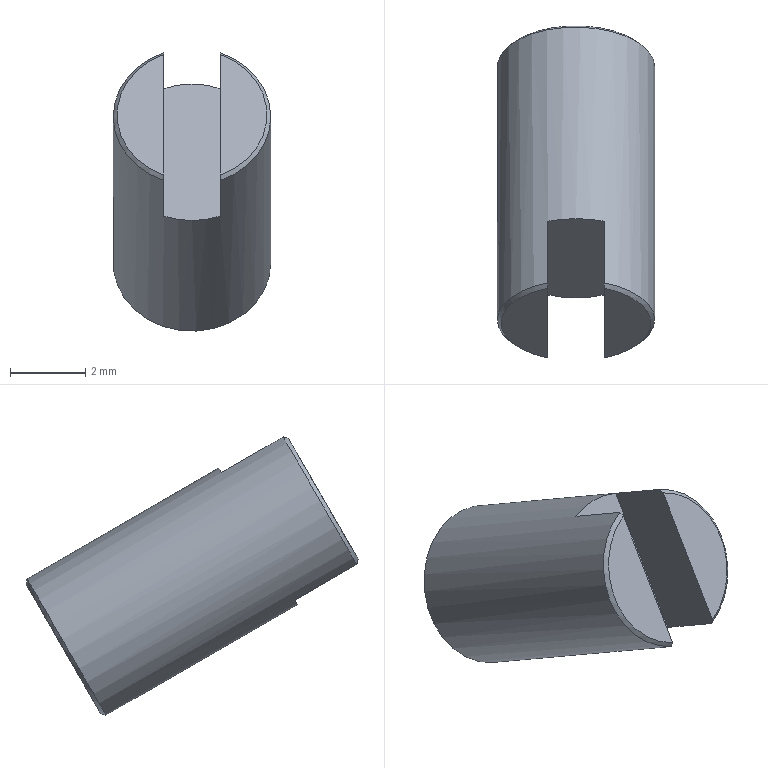Component | NX | 14_AIR_PLUG_2 | 1 solid | 10 faces | box 4.2 x 8.86 x 7.42 mm | volume 98 mm3 | plane 6 | cone 3 | cylinder 1 | commonest cylinder face diameters 4.2 x1
STEP:
#1=CARTESIAN_POINT('',(0.,0.,0.));
#2=DIRECTION('',(0.,0.,1.));
#3=DIRECTION('',(1.,0.,0.));
#4=AXIS2_PLACEMENT_3D('',#1,#2,#3);
#5=CARTESIAN_POINT('',(-58.334,-83.371,-220.899));
#6=VERTEX_POINT('',#5);
#7=CARTESIAN_POINT('',(-58.334,-85.225,-224.111));
#8=VERTEX_POINT('',#7);
#9=CARTESIAN_POINT('',(-58.334,-84.298,-222.505));
#10=DIRECTION('',(0.,-0.5,-0.866));
#11=VECTOR('',#10,1.);
#12=LINE('',#9,#11);
#13=CARTESIAN_POINT('',(-59.084,-84.298,-222.505));
#14=DIRECTION('',(0.,-0.866,0.5));
#15=DIRECTION('',(1.,0.,0.));
#16=AXIS2_PLACEMENT_3D('',#13,#14,#15);
#17=PLANE('',#16);
#18=CARTESIAN_POINT('',(0.75,0.));
#19=DIRECTION('',(0.,-1.));
#20=VECTOR('',#19,1.);
#21=LINE('',#18,#20);
#22=(GEOMETRIC_REPRESENTATION_CONTEXT(2)PARAMETRIC_REPRESENTATION_CONTEXT()REPRESENTATION_CONTEXT('',''));
#23=DEFINITIONAL_REPRESENTATION('',(#21),#22);
#24=PCURVE('',#17,#23);
#25=CARTESIAN_POINT('',(-58.334,-81.316,-221.34));
#26=DIRECTION('',(-1.,-0.,-0.));
#27=DIRECTION('',(0.,-0.5,-0.866));
#28=AXIS2_PLACEMENT_3D('',#25,#26,#27);
#29=PLANE('',#28);
#30=CARTESIAN_POINT('',(2.5,2.));
#31=DIRECTION('',(1.,0.));
#32=VECTOR('',#31,1.);
#33=LINE('',#30,#32);
#34=(GEOMETRIC_REPRESENTATION_CONTEXT(2)PARAMETRIC_REPRESENTATION_CONTEXT()REPRESENTATION_CONTEXT('',''));
#35=DEFINITIONAL_REPRESENTATION('',(#33),#34);
#36=PCURVE('',#29,#35);
#37=SURFACE_CURVE('',#12,(#24,#36),.PCURVE_S1.);
#38=EDGE_CURVE('',#6,#8,#37,.T.);
#39=ORIENTED_EDGE('',*,*,#38,.T.);
#40=CARTESIAN_POINT('',(-59.084,-84.298,-222.505));
#41=DIRECTION('',(0.,-0.866,0.5));
#42=DIRECTION('',(1.,0.,0.));
#43=AXIS2_PLACEMENT_3D('',#40,#41,#42);
#44=CIRCLE('',#43,2.);
#45=CARTESIAN_POINT('',(0.,0.));
#46=DIRECTION('',(1.,0.));
#47=AXIS2_PLACEMENT_2D('',#45,#46);
#48=CIRCLE('',#47,2.);
#49=(GEOMETRIC_REPRESENTATION_CONTEXT(2)PARAMETRIC_REPRESENTATION_CONTEXT()REPRESENTATION_CONTEXT('',''));
#50=DEFINITIONAL_REPRESENTATION('',(#48),#49);
#51=PCURVE('',#17,#50);
#52=CARTESIAN_POINT('',(-59.084,-83.865,-222.755));
#53=DIRECTION('',(0.,0.866,-0.5));
#54=DIRECTION('',(-1.,-0.,-0.));
#55=AXIS2_PLACEMENT_3D('',#52,#53,#54);
#56=CONICAL_SURFACE('',#55,2.5,0.7854);
#57=CARTESIAN_POINT('',(9.425,-0.5));
#58=DIRECTION('',(-1.,-0.));
#59=VECTOR('',#58,1.);
#60=LINE('',#57,#59);
#61=(GEOMETRIC_REPRESENTATION_CONTEXT(2)PARAMETRIC_REPRESENTATION_CONTEXT()REPRESENTATION_CONTEXT('',''));
#62=DEFINITIONAL_REPRESENTATION('',(#60),#61);
#63=PCURVE('',#56,#62);
#64=SURFACE_CURVE('',#44,(#51,#63),.PCURVE_S1.);
#65=EDGE_CURVE('',#8,#6,#64,.T.);
#66=ORIENTED_EDGE('',*,*,#65,.T.);
#67=EDGE_LOOP('',(#39,#66));
#68=FACE_BOUND('',#67,.T.);
#69=ADVANCED_FACE('',(#68),#17,.T.);
#70=CARTESIAN_POINT('',(-59.834,-83.371,-220.899));
#71=VERTEX_POINT('',#70);
#72=CARTESIAN_POINT('',(-59.834,-85.225,-224.111));
#73=VERTEX_POINT('',#72);
#74=CARTESIAN_POINT('',(-59.834,-84.298,-222.505));
#75=DIRECTION('',(0.,-0.5,-0.866));
#76=VECTOR('',#75,1.);
#77=LINE('',#74,#76);
#78=CARTESIAN_POINT('',(-59.084,-84.298,-222.505));
#79=DIRECTION('',(0.,-0.866,0.5));
#80=DIRECTION('',(1.,0.,0.));
#81=AXIS2_PLACEMENT_3D('',#78,#79,#80);
#82=PLANE('',#81);
#83=CARTESIAN_POINT('',(-0.75,0.));
#84=DIRECTION('',(0.,-1.));
#85=VECTOR('',#84,1.);
#86=LINE('',#83,#85);
#87=(GEOMETRIC_REPRESENTATION_CONTEXT(2)PARAMETRIC_REPRESENTATION_CONTEXT()REPRESENTATION_CONTEXT('',''));
#88=DEFINITIONAL_REPRESENTATION('',(#86),#87);
#89=PCURVE('',#82,#88);
#90=CARTESIAN_POINT('',(-59.834,-81.316,-221.34));
#91=DIRECTION('',(-1.,-0.,-0.));
#92=DIRECTION('',(0.,-0.5,-0.866));
#93=AXIS2_PLACEMENT_3D('',#90,#91,#92);
#94=PLANE('',#93);
#95=CARTESIAN_POINT('',(2.5,2.));
#96=DIRECTION('',(1.,0.));
#97=VECTOR('',#96,1.);
#98=LINE('',#95,#97);
#99=(GEOMETRIC_REPRESENTATION_CONTEXT(2)PARAMETRIC_REPRESENTATION_CONTEXT()REPRESENTATION_CONTEXT('',''));
#100=DEFINITIONAL_REPRESENTATION('',(#98),#99);
#101=PCURVE('',#94,#100);
#102=SURFACE_CURVE('',#77,(#89,#101),.PCURVE_S1.);
#103=EDGE_CURVE('',#71,#73,#102,.T.);
#104=ORIENTED_EDGE('',*,*,#103,.F.);
#105=CARTESIAN_POINT('',(-59.084,-84.298,-222.505));
#106=DIRECTION('',(0.,-0.866,0.5));
#107=DIRECTION('',(1.,0.,0.));
#108=AXIS2_PLACEMENT_3D('',#105,#106,#107);
#109=CIRCLE('',#108,2.);
#110=CARTESIAN_POINT('',(0.,0.));
#111=DIRECTION('',(1.,0.));
#112=AXIS2_PLACEMENT_2D('',#110,#111);
#113=CIRCLE('',#112,2.);
#114=(GEOMETRIC_REPRESENTATION_CONTEXT(2)PARAMETRIC_REPRESENTATION_CONTEXT()REPRESENTATION_CONTEXT('',''));
#115=DEFINITIONAL_REPRESENTATION('',(#113),#114);
#116=PCURVE('',#82,#115);
#117=CARTESIAN_POINT('',(-59.084,-83.865,-222.755));
#118=DIRECTION('',(0.,0.866,-0.5));
#119=DIRECTION('',(-1.,-0.,-0.));
#120=AXIS2_PLACEMENT_3D('',#117,#118,#119);
#121=CONICAL_SURFACE('',#120,2.5,0.7854);
#122=CARTESIAN_POINT('',(9.425,-0.5));
#123=DIRECTION('',(-1.,0.));
#124=VECTOR('',#123,1.);
#125=LINE('',#122,#124);
#126=(GEOMETRIC_REPRESENTATION_CONTEXT(2)PARAMETRIC_REPRESENTATION_CONTEXT()REPRESENTATION_CONTEXT('',''));
#127=DEFINITIONAL_REPRESENTATION('',(#125),#126);
#128=PCURVE('',#121,#127);
#129=SURFACE_CURVE('',#109,(#116,#128),.PCURVE_S1.);
#130=EDGE_CURVE('',#71,#73,#129,.T.);
#131=ORIENTED_EDGE('',*,*,#130,.T.);
#132=EDGE_LOOP('',(#104,#131));
#133=FACE_BOUND('',#132,.T.);
#134=ADVANCED_FACE('',(#133),#82,.T.);
#135=CARTESIAN_POINT('',(-61.084,-77.37,-226.505));
#136=VERTEX_POINT('',#135);
#137=CARTESIAN_POINT('',(-57.084,-77.37,-226.505));
#138=VERTEX_POINT('',#137);
#139=CARTESIAN_POINT('',(-59.084,-77.37,-226.505));
#140=DIRECTION('',(0.,0.866,-0.5));
#141=DIRECTION('',(-1.,0.,0.));
#142=AXIS2_PLACEMENT_3D('',#139,#140,#141);
#143=CIRCLE('',#142,2.);
#144=CARTESIAN_POINT('',(-59.084,-77.37,-226.505));
#145=DIRECTION('',(0.,0.866,-0.5));
#146=DIRECTION('',(-1.,0.,0.));
#147=AXIS2_PLACEMENT_3D('',#144,#145,#146);
#148=PLANE('',#147);
#149=CARTESIAN_POINT('',(0.,0.));
#150=DIRECTION('',(1.,0.));
#151=AXIS2_PLACEMENT_2D('',#149,#150);
#152=CIRCLE('',#151,2.);
#153=(GEOMETRIC_REPRESENTATION_CONTEXT(2)PARAMETRIC_REPRESENTATION_CONTEXT()REPRESENTATION_CONTEXT('',''));
#154=DEFINITIONAL_REPRESENTATION('',(#152),#153);
#155=PCURVE('',#148,#154);
#156=CARTESIAN_POINT('',(-59.084,-77.803,-226.255));
#157=DIRECTION('',(0.,-0.866,0.5));
#158=DIRECTION('',(1.,0.,0.));
#159=AXIS2_PLACEMENT_3D('',#156,#157,#158);
#160=CONICAL_SURFACE('',#159,2.5,0.7854);
#161=CARTESIAN_POINT('',(3.142,-0.5));
#162=DIRECTION('',(-1.,0.));
#163=VECTOR('',#162,1.);
#164=LINE('',#161,#163);
#165=(GEOMETRIC_REPRESENTATION_CONTEXT(2)PARAMETRIC_REPRESENTATION_CONTEXT()REPRESENTATION_CONTEXT('',''));
#166=DEFINITIONAL_REPRESENTATION('',(#164),#165);
#167=PCURVE('',#160,#166);
#168=SURFACE_CURVE('',#143,(#155,#167),.PCURVE_S1.);
#169=EDGE_CURVE('',#136,#138,#168,.T.);
#170=ORIENTED_EDGE('',*,*,#169,.T.);
#171=CARTESIAN_POINT('',(-59.084,-77.37,-226.505));
#172=DIRECTION('',(0.,0.866,-0.5));
#173=DIRECTION('',(-1.,0.,0.));
#174=AXIS2_PLACEMENT_3D('',#171,#172,#173);
#175=CIRCLE('',#174,2.);
#176=CARTESIAN_POINT('',(0.,0.));
#177=DIRECTION('',(1.,0.));
#178=AXIS2_PLACEMENT_2D('',#176,#177);
#179=CIRCLE('',#178,2.);
#180=(GEOMETRIC_REPRESENTATION_CONTEXT(2)PARAMETRIC_REPRESENTATION_CONTEXT()REPRESENTATION_CONTEXT('',''));
#181=DEFINITIONAL_REPRESENTATION('',(#179),#180);
#182=PCURVE('',#148,#181);
#183=CARTESIAN_POINT('',(9.425,-0.5));
#184=DIRECTION('',(-1.,0.));
#185=VECTOR('',#184,1.);
#186=LINE('',#183,#185);
#187=(GEOMETRIC_REPRESENTATION_CONTEXT(2)PARAMETRIC_REPRESENTATION_CONTEXT()REPRESENTATION_CONTEXT('',''));
#188=DEFINITIONAL_REPRESENTATION('',(#186),#187);
#189=PCURVE('',#160,#188);
#190=SURFACE_CURVE('',#175,(#182,#189),.PCURVE_S1.);
#191=EDGE_CURVE('',#138,#136,#190,.T.);
#192=ORIENTED_EDGE('',*,*,#191,.T.);
#193=EDGE_LOOP('',(#170,#192));
#194=FACE_BOUND('',#193,.T.);
#195=ADVANCED_FACE('',(#194),#148,.T.);
#196=CARTESIAN_POINT('',(-56.984,-77.457,-226.455));
#197=VERTEX_POINT('',#196);
#198=CARTESIAN_POINT('',(-59.084,-77.457,-226.455));
#199=DIRECTION('',(0.,-0.866,0.5));
#200=DIRECTION('',(1.,0.,0.));
#201=AXIS2_PLACEMENT_3D('',#198,#199,#200);
#202=CIRCLE('',#201,2.1);
#203=CARTESIAN_POINT('',(-59.084,-77.37,-226.505));
#204=DIRECTION('',(0.,-0.866,0.5));
#205=DIRECTION('',(1.,0.,0.));
#206=AXIS2_PLACEMENT_3D('',#203,#204,#205);
#207=CYLINDRICAL_SURFACE('',#206,2.1);
#208=CARTESIAN_POINT('',(0.,0.1));
#209=DIRECTION('',(1.,0.));
#210=VECTOR('',#209,1.);
#211=LINE('',#208,#210);
#212=(GEOMETRIC_REPRESENTATION_CONTEXT(2)PARAMETRIC_REPRESENTATION_CONTEXT()REPRESENTATION_CONTEXT('',''));
#213=DEFINITIONAL_REPRESENTATION('',(#211),#212);
#214=PCURVE('',#207,#213);
#215=CARTESIAN_POINT('',(0.,-0.4));
#216=DIRECTION('',(1.,0.));
#217=VECTOR('',#216,1.);
#218=LINE('',#215,#217);
#219=(GEOMETRIC_REPRESENTATION_CONTEXT(2)PARAMETRIC_REPRESENTATION_CONTEXT()REPRESENTATION_CONTEXT('',''));
#220=DEFINITIONAL_REPRESENTATION('',(#218),#219);
#221=PCURVE('',#160,#220);
#222=SURFACE_CURVE('',#202,(#214,#221),.PCURVE_S1.);
#223=EDGE_CURVE('',#197,#197,#222,.T.);
#224=ORIENTED_EDGE('',*,*,#223,.T.);
#225=CARTESIAN_POINT('',(-56.984,-84.212,-222.555));
#226=VERTEX_POINT('',#225);
#227=CARTESIAN_POINT('',(-56.984,-77.457,-226.455));
#228=CARTESIAN_POINT('',(-56.984,-84.212,-222.555));
#229=B_SPLINE_CURVE_WITH_KNOTS('',1,(#227,#228),.UNSPECIFIED.,.F.,.F.,(2,2),(0.1,7.9),.PIECEWISE_BEZIER_KNOTS.);
#230=CARTESIAN_POINT('',(6.283,0.));
#231=DIRECTION('',(0.,1.));
#232=VECTOR('',#231,1.);
#233=LINE('',#230,#232);
#234=(GEOMETRIC_REPRESENTATION_CONTEXT(2)PARAMETRIC_REPRESENTATION_CONTEXT()REPRESENTATION_CONTEXT('',''));
#235=DEFINITIONAL_REPRESENTATION('',(#233),#234);
#236=PCURVE('',#207,#235);
#237=CARTESIAN_POINT('',(0.,0.));
#238=DIRECTION('',(0.,1.));
#239=VECTOR('',#238,1.);
#240=LINE('',#237,#239);
#241=(GEOMETRIC_REPRESENTATION_CONTEXT(2)PARAMETRIC_REPRESENTATION_CONTEXT()REPRESENTATION_CONTEXT('',''));
#242=DEFINITIONAL_REPRESENTATION('',(#240),#241);
#243=PCURVE('',#207,#242);
#244=SEAM_CURVE('',#229,(#236,#243),.PCURVE_S1.);
#245=EDGE_CURVE('',#197,#226,#244,.T.);
#246=ORIENTED_EDGE('',*,*,#245,.T.);
#247=CARTESIAN_POINT('',(-58.334,-85.193,-224.254));
#248=VERTEX_POINT('',#247);
#249=CARTESIAN_POINT('',(-59.084,-84.212,-222.555));
#250=DIRECTION('',(0.,0.866,-0.5));
#251=DIRECTION('',(-1.,0.,0.));
#252=AXIS2_PLACEMENT_3D('',#249,#250,#251);
#253=CIRCLE('',#252,2.1);
#254=CARTESIAN_POINT('',(9.425,7.9));
#255=DIRECTION('',(-1.,-0.));
#256=VECTOR('',#255,1.);
#257=LINE('',#254,#256);
#258=(GEOMETRIC_REPRESENTATION_CONTEXT(2)PARAMETRIC_REPRESENTATION_CONTEXT()REPRESENTATION_CONTEXT('',''));
#259=DEFINITIONAL_REPRESENTATION('',(#257),#258);
#260=PCURVE('',#207,#259);
#261=CARTESIAN_POINT('',(0.,-0.4));
#262=DIRECTION('',(1.,0.));
#263=VECTOR('',#262,1.);
#264=LINE('',#261,#263);
#265=(GEOMETRIC_REPRESENTATION_CONTEXT(2)PARAMETRIC_REPRESENTATION_CONTEXT()REPRESENTATION_CONTEXT('',''));
#266=DEFINITIONAL_REPRESENTATION('',(#264),#265);
#267=PCURVE('',#56,#266);
#268=SURFACE_CURVE('',#253,(#260,#267),.PCURVE_S1.);
#269=EDGE_CURVE('',#226,#248,#268,.T.);
#270=ORIENTED_EDGE('',*,*,#269,.T.);
#271=CARTESIAN_POINT('',(-58.334,-83.547,-225.204));
#272=VERTEX_POINT('',#271);
#273=CARTESIAN_POINT('',(-58.334,-78.351,-228.204));
#274=DIRECTION('',(0.,0.866,-0.5));
#275=VECTOR('',#274,1.);
#276=LINE('',#273,#275);
#277=CARTESIAN_POINT('',(5.078,-0.));
#278=DIRECTION('',(0.,-1.));
#279=VECTOR('',#278,1.);
#280=LINE('',#277,#279);
#281=(GEOMETRIC_REPRESENTATION_CONTEXT(2)PARAMETRIC_REPRESENTATION_CONTEXT()REPRESENTATION_CONTEXT('',''));
#282=DEFINITIONAL_REPRESENTATION('',(#280),#281);
#283=PCURVE('',#207,#282);
#284=CARTESIAN_POINT('',(4.462,-6.));
#285=DIRECTION('',(0.,-1.));
#286=VECTOR('',#285,1.);
#287=LINE('',#284,#286);
#288=(GEOMETRIC_REPRESENTATION_CONTEXT(2)PARAMETRIC_REPRESENTATION_CONTEXT()REPRESENTATION_CONTEXT('',''));
#289=DEFINITIONAL_REPRESENTATION('',(#287),#288);
#290=PCURVE('',#29,#289);
#291=SURFACE_CURVE('',#276,(#283,#290),.PCURVE_S1.);
#292=EDGE_CURVE('',#248,#272,#291,.T.);
#293=ORIENTED_EDGE('',*,*,#292,.T.);
#294=CARTESIAN_POINT('',(-59.834,-83.547,-225.204));
#295=VERTEX_POINT('',#294);
#296=CARTESIAN_POINT('',(-59.084,-82.566,-223.505));
#297=DIRECTION('',(0.,-0.866,0.5));
#298=DIRECTION('',(-1.,0.,0.));
#299=AXIS2_PLACEMENT_3D('',#296,#297,#298);
#300=CIRCLE('',#299,2.1);
#301=CARTESIAN_POINT('',(3.142,6.));
#302=DIRECTION('',(1.,0.));
#303=VECTOR('',#302,1.);
#304=LINE('',#301,#303);
#305=(GEOMETRIC_REPRESENTATION_CONTEXT(2)PARAMETRIC_REPRESENTATION_CONTEXT()REPRESENTATION_CONTEXT('',''));
#306=DEFINITIONAL_REPRESENTATION('',(#304),#305);
#307=PCURVE('',#207,#306);
#308=CARTESIAN_POINT('',(-59.084,-81.316,-221.34));
#309=DIRECTION('',(0.,0.866,-0.5));
#310=DIRECTION('',(0.,-0.5,-0.866));
#311=AXIS2_PLACEMENT_3D('',#308,#309,#310);
#312=PLANE('',#311);
#313=CARTESIAN_POINT('',(2.5,2.1));
#314=CARTESIAN_POINT('',(6.137,2.1));
#315=CARTESIAN_POINT('',(4.319,-1.05));
#316=CARTESIAN_POINT('',(2.5,-4.2));
#317=CARTESIAN_POINT('',(0.6813,-1.05));
#318=CARTESIAN_POINT('',(-1.137,2.1));
#319=CARTESIAN_POINT('',(2.5,2.1));
#320=(BOUNDED_CURVE()B_SPLINE_CURVE(2,(#313,#314,#315,#316,#317,#318,#319),.UNSPECIFIED.,.T.,.F.)B_SPLINE_CURVE_WITH_KNOTS((1,2,2,2,2,1),(-2.094,0.,2.094,4.189,6.283,8.378),.UNSPECIFIED.)CURVE()GEOMETRIC_REPRESENTATION_ITEM()RATIONAL_B_SPLINE_CURVE((1.,0.5,1.,0.5,1.,0.5,1.))REPRESENTATION_ITEM(''));
#321=(GEOMETRIC_REPRESENTATION_CONTEXT(2)PARAMETRIC_REPRESENTATION_CONTEXT()REPRESENTATION_CONTEXT('',''));
#322=DEFINITIONAL_REPRESENTATION('',(#320),#321);
#323=PCURVE('',#312,#322);
#324=SURFACE_CURVE('',#300,(#307,#323),.PCURVE_S1.);
#325=EDGE_CURVE('',#295,#272,#324,.T.);
#326=ORIENTED_EDGE('',*,*,#325,.F.);
#327=CARTESIAN_POINT('',(-59.834,-85.193,-224.254));
#328=VERTEX_POINT('',#327);
#329=CARTESIAN_POINT('',(-59.834,-78.351,-228.204));
#330=DIRECTION('',(0.,0.866,-0.5));
#331=VECTOR('',#330,1.);
#332=LINE('',#329,#331);
#333=CARTESIAN_POINT('',(4.347,-0.));
#334=DIRECTION('',(0.,-1.));
#335=VECTOR('',#334,1.);
#336=LINE('',#333,#335);
#337=(GEOMETRIC_REPRESENTATION_CONTEXT(2)PARAMETRIC_REPRESENTATION_CONTEXT()REPRESENTATION_CONTEXT('',''));
#338=DEFINITIONAL_REPRESENTATION('',(#336),#337);
#339=PCURVE('',#207,#338);
#340=CARTESIAN_POINT('',(4.462,-6.));
#341=DIRECTION('',(0.,-1.));
#342=VECTOR('',#341,1.);
#343=LINE('',#340,#342);
#344=(GEOMETRIC_REPRESENTATION_CONTEXT(2)PARAMETRIC_REPRESENTATION_CONTEXT()REPRESENTATION_CONTEXT('',''));
#345=DEFINITIONAL_REPRESENTATION('',(#343),#344);
#346=PCURVE('',#94,#345);
#347=SURFACE_CURVE('',#332,(#339,#346),.PCURVE_S1.);
#348=EDGE_CURVE('',#328,#295,#347,.T.);
#349=ORIENTED_EDGE('',*,*,#348,.F.);
#350=CARTESIAN_POINT('',(-59.834,-83.231,-220.856));
#351=VERTEX_POINT('',#350);
#352=CARTESIAN_POINT('',(-59.084,-84.212,-222.555));
#353=DIRECTION('',(0.,0.866,-0.5));
#354=DIRECTION('',(-1.,0.,0.));
#355=AXIS2_PLACEMENT_3D('',#352,#353,#354);
#356=CIRCLE('',#355,2.1);
#357=CARTESIAN_POINT('',(9.425,7.9));
#358=DIRECTION('',(-1.,0.));
#359=VECTOR('',#358,1.);
#360=LINE('',#357,#359);
#361=(GEOMETRIC_REPRESENTATION_CONTEXT(2)PARAMETRIC_REPRESENTATION_CONTEXT()REPRESENTATION_CONTEXT('',''));
#362=DEFINITIONAL_REPRESENTATION('',(#360),#361);
#363=PCURVE('',#207,#362);
#364=CARTESIAN_POINT('',(-0.,-0.4));
#365=DIRECTION('',(1.,-0.));
#366=VECTOR('',#365,1.);
#367=LINE('',#364,#366);
#368=(GEOMETRIC_REPRESENTATION_CONTEXT(2)PARAMETRIC_REPRESENTATION_CONTEXT()REPRESENTATION_CONTEXT('',''));
#369=DEFINITIONAL_REPRESENTATION('',(#367),#368);
#370=PCURVE('',#121,#369);
#371=SURFACE_CURVE('',#356,(#363,#370),.PCURVE_S1.);
#372=EDGE_CURVE('',#328,#351,#371,.T.);
#373=ORIENTED_EDGE('',*,*,#372,.T.);
#374=CARTESIAN_POINT('',(-59.834,-81.586,-221.806));
#375=VERTEX_POINT('',#374);
#376=CARTESIAN_POINT('',(-59.834,-76.389,-224.806));
#377=DIRECTION('',(0.,-0.866,0.5));
#378=VECTOR('',#377,1.);
#379=LINE('',#376,#378);
#380=CARTESIAN_POINT('',(1.936,-0.));
#381=DIRECTION('',(0.,1.));
#382=VECTOR('',#381,1.);
#383=LINE('',#380,#382);
#384=(GEOMETRIC_REPRESENTATION_CONTEXT(2)PARAMETRIC_REPRESENTATION_CONTEXT()REPRESENTATION_CONTEXT('',''));
#385=DEFINITIONAL_REPRESENTATION('',(#383),#384);
#386=PCURVE('',#207,#385);
#387=CARTESIAN_POINT('',(0.5385,-6.));
#388=DIRECTION('',(0.,1.));
#389=VECTOR('',#388,1.);
#390=LINE('',#387,#389);
#391=(GEOMETRIC_REPRESENTATION_CONTEXT(2)PARAMETRIC_REPRESENTATION_CONTEXT()REPRESENTATION_CONTEXT('',''));
#392=DEFINITIONAL_REPRESENTATION('',(#390),#391);
#393=PCURVE('',#94,#392);
#394=SURFACE_CURVE('',#379,(#386,#393),.PCURVE_S1.);
#395=EDGE_CURVE('',#375,#351,#394,.T.);
#396=ORIENTED_EDGE('',*,*,#395,.F.);
#397=CARTESIAN_POINT('',(-58.334,-81.586,-221.806));
#398=VERTEX_POINT('',#397);
#399=CARTESIAN_POINT('',(-59.084,-82.566,-223.505));
#400=DIRECTION('',(0.,-0.866,0.5));
#401=DIRECTION('',(-1.,0.,0.));
#402=AXIS2_PLACEMENT_3D('',#399,#400,#401);
#403=CIRCLE('',#402,2.1);
#404=CARTESIAN_POINT('',(-3.142,6.));
#405=DIRECTION('',(1.,0.));
#406=VECTOR('',#405,1.);
#407=LINE('',#404,#406);
#408=(GEOMETRIC_REPRESENTATION_CONTEXT(2)PARAMETRIC_REPRESENTATION_CONTEXT()REPRESENTATION_CONTEXT('',''));
#409=DEFINITIONAL_REPRESENTATION('',(#407),#408);
#410=PCURVE('',#207,#409);
#411=CARTESIAN_POINT('',(2.5,2.1));
#412=CARTESIAN_POINT('',(6.137,2.1));
#413=CARTESIAN_POINT('',(4.319,-1.05));
#414=CARTESIAN_POINT('',(2.5,-4.2));
#415=CARTESIAN_POINT('',(0.6813,-1.05));
#416=CARTESIAN_POINT('',(-1.137,2.1));
#417=CARTESIAN_POINT('',(2.5,2.1));
#418=(BOUNDED_CURVE()B_SPLINE_CURVE(2,(#411,#412,#413,#414,#415,#416,#417),.UNSPECIFIED.,.T.,.F.)B_SPLINE_CURVE_WITH_KNOTS((1,2,2,2,2,1),(-2.094,0.,2.094,4.189,6.283,8.378),.UNSPECIFIED.)CURVE()GEOMETRIC_REPRESENTATION_ITEM()RATIONAL_B_SPLINE_CURVE((1.,0.5,1.,0.5,1.,0.5,1.))REPRESENTATION_ITEM(''));
#419=(GEOMETRIC_REPRESENTATION_CONTEXT(2)PARAMETRIC_REPRESENTATION_CONTEXT()REPRESENTATION_CONTEXT('',''));
#420=DEFINITIONAL_REPRESENTATION('',(#418),#419);
#421=PCURVE('',#312,#420);
#422=SURFACE_CURVE('',#403,(#410,#421),.PCURVE_S1.);
#423=EDGE_CURVE('',#398,#375,#422,.T.);
#424=ORIENTED_EDGE('',*,*,#423,.F.);
#425=CARTESIAN_POINT('',(-58.334,-83.231,-220.856));
#426=VERTEX_POINT('',#425);
#427=CARTESIAN_POINT('',(-58.334,-76.389,-224.806));
#428=DIRECTION('',(0.,-0.866,0.5));
#429=VECTOR('',#428,1.);
#430=LINE('',#427,#429);
#431=CARTESIAN_POINT('',(1.206,-0.));
#432=DIRECTION('',(0.,1.));
#433=VECTOR('',#432,1.);
#434=LINE('',#431,#433);
#435=(GEOMETRIC_REPRESENTATION_CONTEXT(2)PARAMETRIC_REPRESENTATION_CONTEXT()REPRESENTATION_CONTEXT('',''));
#436=DEFINITIONAL_REPRESENTATION('',(#434),#435);
#437=PCURVE('',#207,#436);
#438=CARTESIAN_POINT('',(0.5385,-6.));
#439=DIRECTION('',(0.,1.));
#440=VECTOR('',#439,1.);
#441=LINE('',#438,#440);
#442=(GEOMETRIC_REPRESENTATION_CONTEXT(2)PARAMETRIC_REPRESENTATION_CONTEXT()REPRESENTATION_CONTEXT('',''));
#443=DEFINITIONAL_REPRESENTATION('',(#441),#442);
#444=PCURVE('',#29,#443);
#445=SURFACE_CURVE('',#430,(#437,#444),.PCURVE_S1.);
#446=EDGE_CURVE('',#398,#426,#445,.T.);
#447=ORIENTED_EDGE('',*,*,#446,.T.);
#448=CARTESIAN_POINT('',(-59.084,-84.212,-222.555));
#449=DIRECTION('',(0.,0.866,-0.5));
#450=DIRECTION('',(-1.,0.,0.));
#451=AXIS2_PLACEMENT_3D('',#448,#449,#450);
#452=CIRCLE('',#451,2.1);
#453=CARTESIAN_POINT('',(3.142,7.9));
#454=DIRECTION('',(-1.,-0.));
#455=VECTOR('',#454,1.);
#456=LINE('',#453,#455);
#457=(GEOMETRIC_REPRESENTATION_CONTEXT(2)PARAMETRIC_REPRESENTATION_CONTEXT()REPRESENTATION_CONTEXT('',''));
#458=DEFINITIONAL_REPRESENTATION('',(#456),#457);
#459=PCURVE('',#207,#458);
#460=CARTESIAN_POINT('',(0.,-0.4));
#461=DIRECTION('',(1.,0.));
#462=VECTOR('',#461,1.);
#463=LINE('',#460,#462);
#464=(GEOMETRIC_REPRESENTATION_CONTEXT(2)PARAMETRIC_REPRESENTATION_CONTEXT()REPRESENTATION_CONTEXT('',''));
#465=DEFINITIONAL_REPRESENTATION('',(#463),#464);
#466=PCURVE('',#56,#465);
#467=SURFACE_CURVE('',#452,(#459,#466),.PCURVE_S1.);
#468=EDGE_CURVE('',#426,#226,#467,.T.);
#469=ORIENTED_EDGE('',*,*,#468,.T.);
#470=ORIENTED_EDGE('',*,*,#245,.F.);
#471=EDGE_LOOP('',(#224,#246,#270,#293,#326,#349,#373,#396,#424,#447,#469,#470));
#472=FACE_BOUND('',#471,.T.);
#473=ADVANCED_FACE('',(#472),#207,.T.);
#474=CARTESIAN_POINT('',(-59.834,-81.316,-221.34));
#475=DIRECTION('',(-0.,0.5,0.866));
#476=VECTOR('',#475,1.);
#477=LINE('',#474,#476);
#478=CARTESIAN_POINT('',(-0.,0.75));
#479=DIRECTION('',(-1.,-0.));
#480=VECTOR('',#479,1.);
#481=LINE('',#478,#480);
#482=(GEOMETRIC_REPRESENTATION_CONTEXT(2)PARAMETRIC_REPRESENTATION_CONTEXT()REPRESENTATION_CONTEXT('',''));
#483=DEFINITIONAL_REPRESENTATION('',(#481),#482);
#484=PCURVE('',#312,#483);
#485=CARTESIAN_POINT('',(0.,0.));
#486=DIRECTION('',(-1.,0.));
#487=VECTOR('',#486,1.);
#488=LINE('',#485,#487);
#489=(GEOMETRIC_REPRESENTATION_CONTEXT(2)PARAMETRIC_REPRESENTATION_CONTEXT()REPRESENTATION_CONTEXT('',''));
#490=DEFINITIONAL_REPRESENTATION('',(#488),#489);
#491=PCURVE('',#94,#490);
#492=SURFACE_CURVE('',#477,(#484,#491),.PCURVE_S1.);
#493=EDGE_CURVE('',#295,#375,#492,.T.);
#494=ORIENTED_EDGE('',*,*,#493,.F.);
#495=ORIENTED_EDGE('',*,*,#325,.T.);
#496=CARTESIAN_POINT('',(-58.334,-81.316,-221.34));
#497=DIRECTION('',(-0.,0.5,0.866));
#498=VECTOR('',#497,1.);
#499=LINE('',#496,#498);
#500=CARTESIAN_POINT('',(0.,-0.75));
#501=DIRECTION('',(-1.,-0.));
#502=VECTOR('',#501,1.);
#503=LINE('',#500,#502);
#504=(GEOMETRIC_REPRESENTATION_CONTEXT(2)PARAMETRIC_REPRESENTATION_CONTEXT()REPRESENTATION_CONTEXT('',''));
#505=DEFINITIONAL_REPRESENTATION('',(#503),#504);
#506=PCURVE('',#312,#505);
#507=CARTESIAN_POINT('',(0.,0.));
#508=DIRECTION('',(-1.,0.));
#509=VECTOR('',#508,1.);
#510=LINE('',#507,#509);
#511=(GEOMETRIC_REPRESENTATION_CONTEXT(2)PARAMETRIC_REPRESENTATION_CONTEXT()REPRESENTATION_CONTEXT('',''));
#512=DEFINITIONAL_REPRESENTATION('',(#510),#511);
#513=PCURVE('',#29,#512);
#514=SURFACE_CURVE('',#499,(#506,#513),.PCURVE_S1.);
#515=EDGE_CURVE('',#272,#398,#514,.T.);
#516=ORIENTED_EDGE('',*,*,#515,.T.);
#517=ORIENTED_EDGE('',*,*,#423,.T.);
#518=EDGE_LOOP('',(#494,#495,#516,#517));
#519=FACE_BOUND('',#518,.T.);
#520=ADVANCED_FACE('',(#519),#312,.F.);
#521=ORIENTED_EDGE('',*,*,#395,.T.);
#522=CARTESIAN_POINT('',(-59.834,-83.231,-220.856));
#523=CARTESIAN_POINT('',(-59.834,-83.278,-220.87));
#524=CARTESIAN_POINT('',(-59.834,-83.325,-220.885));
#525=CARTESIAN_POINT('',(-59.834,-83.371,-220.899));
#526=B_SPLINE_CURVE_WITH_KNOTS('',3,(#522,#523,#524,#525),.UNSPECIFIED.,.F.,.F.,(4,4),(0.,1.),.PIECEWISE_BEZIER_KNOTS.);
#527=CARTESIAN_POINT('',(0.5385,1.9));
#528=CARTESIAN_POINT('',(0.5743,1.933));
#529=CARTESIAN_POINT('',(0.6101,1.967));
#530=CARTESIAN_POINT('',(0.646,2.));
#531=B_SPLINE_CURVE_WITH_KNOTS('',3,(#527,#528,#529,#530),.UNSPECIFIED.,.F.,.F.,(4,4),(0.,1.),.PIECEWISE_BEZIER_KNOTS.);
#532=(GEOMETRIC_REPRESENTATION_CONTEXT(2)PARAMETRIC_REPRESENTATION_CONTEXT()REPRESENTATION_CONTEXT('',''));
#533=DEFINITIONAL_REPRESENTATION('',(#531),#532);
#534=PCURVE('',#94,#533);
#535=CARTESIAN_POINT('',(7.489,-0.4));
#536=CARTESIAN_POINT('',(7.47,-0.5));
#537=B_SPLINE_CURVE_WITH_KNOTS('',1,(#535,#536),.UNSPECIFIED.,.F.,.F.,(2,2),(0.,1.),.PIECEWISE_BEZIER_KNOTS.);
#538=(GEOMETRIC_REPRESENTATION_CONTEXT(2)PARAMETRIC_REPRESENTATION_CONTEXT()REPRESENTATION_CONTEXT('',''));
#539=DEFINITIONAL_REPRESENTATION('',(#537),#538);
#540=PCURVE('',#121,#539);
#541=SURFACE_CURVE('',#526,(#534,#540),.PCURVE_S1.);
#542=EDGE_CURVE('',#351,#71,#541,.T.);
#543=ORIENTED_EDGE('',*,*,#542,.T.);
#544=ORIENTED_EDGE('',*,*,#103,.T.);
#545=CARTESIAN_POINT('',(-59.834,-85.225,-224.111));
#546=CARTESIAN_POINT('',(-59.834,-85.215,-224.158));
#547=CARTESIAN_POINT('',(-59.834,-85.204,-224.206));
#548=CARTESIAN_POINT('',(-59.834,-85.193,-224.254));
#549=B_SPLINE_CURVE_WITH_KNOTS('',3,(#545,#546,#547,#548),.UNSPECIFIED.,.F.,.F.,(4,4),(0.,1.),.PIECEWISE_BEZIER_KNOTS.);
#550=CARTESIAN_POINT('',(4.354,2.));
#551=CARTESIAN_POINT('',(4.39,1.967));
#552=CARTESIAN_POINT('',(4.426,1.933));
#553=CARTESIAN_POINT('',(4.462,1.9));
#554=B_SPLINE_CURVE_WITH_KNOTS('',3,(#550,#551,#552,#553),.UNSPECIFIED.,.F.,.F.,(4,4),(0.,1.),.PIECEWISE_BEZIER_KNOTS.);
#555=(GEOMETRIC_REPRESENTATION_CONTEXT(2)PARAMETRIC_REPRESENTATION_CONTEXT()REPRESENTATION_CONTEXT('',''));
#556=DEFINITIONAL_REPRESENTATION('',(#554),#555);
#557=PCURVE('',#94,#556);
#558=CARTESIAN_POINT('',(5.097,-0.5));
#559=CARTESIAN_POINT('',(5.078,-0.4));
#560=B_SPLINE_CURVE_WITH_KNOTS('',1,(#558,#559),.UNSPECIFIED.,.F.,.F.,(2,2),(0.,1.),.PIECEWISE_BEZIER_KNOTS.);
#561=(GEOMETRIC_REPRESENTATION_CONTEXT(2)PARAMETRIC_REPRESENTATION_CONTEXT()REPRESENTATION_CONTEXT('',''));
#562=DEFINITIONAL_REPRESENTATION('',(#560),#561);
#563=PCURVE('',#121,#562);
#564=SURFACE_CURVE('',#549,(#557,#563),.PCURVE_S1.);
#565=EDGE_CURVE('',#73,#328,#564,.T.);
#566=ORIENTED_EDGE('',*,*,#565,.T.);
#567=ORIENTED_EDGE('',*,*,#348,.T.);
#568=ORIENTED_EDGE('',*,*,#493,.T.);
#569=EDGE_LOOP('',(#521,#543,#544,#566,#567,#568));
#570=FACE_BOUND('',#569,.T.);
#571=ADVANCED_FACE('',(#570),#94,.F.);
#572=ORIENTED_EDGE('',*,*,#292,.F.);
#573=CARTESIAN_POINT('',(-58.334,-85.193,-224.254));
#574=CARTESIAN_POINT('',(-58.334,-85.204,-224.206));
#575=CARTESIAN_POINT('',(-58.334,-85.215,-224.158));
#576=CARTESIAN_POINT('',(-58.334,-85.225,-224.111));
#577=B_SPLINE_CURVE_WITH_KNOTS('',3,(#573,#574,#575,#576),.UNSPECIFIED.,.F.,.F.,(4,4),(0.,1.),.PIECEWISE_BEZIER_KNOTS.);
#578=CARTESIAN_POINT('',(4.462,1.9));
#579=CARTESIAN_POINT('',(4.426,1.933));
#580=CARTESIAN_POINT('',(4.39,1.967));
#581=CARTESIAN_POINT('',(4.354,2.));
#582=B_SPLINE_CURVE_WITH_KNOTS('',3,(#578,#579,#580,#581),.UNSPECIFIED.,.F.,.F.,(4,4),(0.,1.),.PIECEWISE_BEZIER_KNOTS.);
#583=(GEOMETRIC_REPRESENTATION_CONTEXT(2)PARAMETRIC_REPRESENTATION_CONTEXT()REPRESENTATION_CONTEXT('',''));
#584=DEFINITIONAL_REPRESENTATION('',(#582),#583);
#585=PCURVE('',#29,#584);
#586=CARTESIAN_POINT('',(4.347,-0.4));
#587=CARTESIAN_POINT('',(4.328,-0.5));
#588=B_SPLINE_CURVE_WITH_KNOTS('',1,(#586,#587),.UNSPECIFIED.,.F.,.F.,(2,2),(0.,1.),.PIECEWISE_BEZIER_KNOTS.);
#589=(GEOMETRIC_REPRESENTATION_CONTEXT(2)PARAMETRIC_REPRESENTATION_CONTEXT()REPRESENTATION_CONTEXT('',''));
#590=DEFINITIONAL_REPRESENTATION('',(#588),#589);
#591=PCURVE('',#56,#590);
#592=SURFACE_CURVE('',#577,(#585,#591),.PCURVE_S1.);
#593=EDGE_CURVE('',#248,#8,#592,.T.);
#594=ORIENTED_EDGE('',*,*,#593,.T.);
#595=ORIENTED_EDGE('',*,*,#38,.F.);
#596=CARTESIAN_POINT('',(-58.334,-83.371,-220.899));
#597=CARTESIAN_POINT('',(-58.334,-83.325,-220.885));
#598=CARTESIAN_POINT('',(-58.334,-83.278,-220.87));
#599=CARTESIAN_POINT('',(-58.334,-83.231,-220.856));
#600=B_SPLINE_CURVE_WITH_KNOTS('',3,(#596,#597,#598,#599),.UNSPECIFIED.,.F.,.F.,(4,4),(0.,1.),.PIECEWISE_BEZIER_KNOTS.);
#601=CARTESIAN_POINT('',(0.646,2.));
#602=CARTESIAN_POINT('',(0.6101,1.967));
#603=CARTESIAN_POINT('',(0.5743,1.933));
#604=CARTESIAN_POINT('',(0.5385,1.9));
#605=B_SPLINE_CURVE_WITH_KNOTS('',3,(#601,#602,#603,#604),.UNSPECIFIED.,.F.,.F.,(4,4),(0.,1.),.PIECEWISE_BEZIER_KNOTS.);
#606=(GEOMETRIC_REPRESENTATION_CONTEXT(2)PARAMETRIC_REPRESENTATION_CONTEXT()REPRESENTATION_CONTEXT('',''));
#607=DEFINITIONAL_REPRESENTATION('',(#605),#606);
#608=PCURVE('',#29,#607);
#609=CARTESIAN_POINT('',(1.955,-0.5));
#610=CARTESIAN_POINT('',(1.936,-0.4));
#611=B_SPLINE_CURVE_WITH_KNOTS('',1,(#609,#610),.UNSPECIFIED.,.F.,.F.,(2,2),(0.,1.),.PIECEWISE_BEZIER_KNOTS.);
#612=(GEOMETRIC_REPRESENTATION_CONTEXT(2)PARAMETRIC_REPRESENTATION_CONTEXT()REPRESENTATION_CONTEXT('',''));
#613=DEFINITIONAL_REPRESENTATION('',(#611),#612);
#614=PCURVE('',#56,#613);
#615=SURFACE_CURVE('',#600,(#608,#614),.PCURVE_S1.);
#616=EDGE_CURVE('',#6,#426,#615,.T.);
#617=ORIENTED_EDGE('',*,*,#616,.T.);
#618=ORIENTED_EDGE('',*,*,#446,.F.);
#619=ORIENTED_EDGE('',*,*,#515,.F.);
#620=EDGE_LOOP('',(#572,#594,#595,#617,#618,#619));
#621=FACE_BOUND('',#620,.T.);
#622=ADVANCED_FACE('',(#621),#29,.T.);
#623=ORIENTED_EDGE('',*,*,#191,.F.);
#624=CARTESIAN_POINT('',(-57.084,-77.37,-226.505));
#625=CARTESIAN_POINT('',(-56.984,-77.457,-226.455));
#626=B_SPLINE_CURVE_WITH_KNOTS('',1,(#624,#625),.UNSPECIFIED.,.F.,.F.,(2,2),(-0.7071,-0.5657),.PIECEWISE_BEZIER_KNOTS.);
#627=CARTESIAN_POINT('',(6.283,0.));
#628=DIRECTION('',(0.,1.));
#629=VECTOR('',#628,1.);
#630=LINE('',#627,#629);
#631=(GEOMETRIC_REPRESENTATION_CONTEXT(2)PARAMETRIC_REPRESENTATION_CONTEXT()REPRESENTATION_CONTEXT('',''));
#632=DEFINITIONAL_REPRESENTATION('',(#630),#631);
#633=PCURVE('',#160,#632);
#634=CARTESIAN_POINT('',(0.,0.));
#635=DIRECTION('',(0.,1.));
#636=VECTOR('',#635,1.);
#637=LINE('',#634,#636);
#638=(GEOMETRIC_REPRESENTATION_CONTEXT(2)PARAMETRIC_REPRESENTATION_CONTEXT()REPRESENTATION_CONTEXT('',''));
#639=DEFINITIONAL_REPRESENTATION('',(#637),#638);
#640=PCURVE('',#160,#639);
#641=SEAM_CURVE('',#626,(#633,#640),.PCURVE_S1.);
#642=EDGE_CURVE('',#138,#197,#641,.T.);
#643=ORIENTED_EDGE('',*,*,#642,.T.);
#644=ORIENTED_EDGE('',*,*,#223,.F.);
#645=ORIENTED_EDGE('',*,*,#642,.F.);
#646=ORIENTED_EDGE('',*,*,#169,.F.);
#647=EDGE_LOOP('',(#623,#643,#644,#645,#646));
#648=FACE_BOUND('',#647,.T.);
#649=ADVANCED_FACE('',(#648),#160,.T.);
#650=ORIENTED_EDGE('',*,*,#616,.F.);
#651=ORIENTED_EDGE('',*,*,#65,.F.);
#652=ORIENTED_EDGE('',*,*,#593,.F.);
#653=ORIENTED_EDGE('',*,*,#269,.F.);
#654=ORIENTED_EDGE('',*,*,#468,.F.);
#655=EDGE_LOOP('',(#650,#651,#652,#653,#654));
#656=FACE_BOUND('',#655,.T.);
#657=ADVANCED_FACE('',(#656),#56,.T.);
#658=ORIENTED_EDGE('',*,*,#565,.F.);
#659=ORIENTED_EDGE('',*,*,#130,.F.);
#660=ORIENTED_EDGE('',*,*,#542,.F.);
#661=ORIENTED_EDGE('',*,*,#372,.F.);
#662=EDGE_LOOP('',(#658,#659,#660,#661));
#663=FACE_BOUND('',#662,.T.);
#664=ADVANCED_FACE('',(#663),#121,.T.);
#665=CLOSED_SHELL('',(#69,#134,#195,#473,#520,#571,#622,#649,#657,#664));
#666=MANIFOLD_SOLID_BREP('',#665);
#667=(LENGTH_UNIT()NAMED_UNIT(*)SI_UNIT(.MILLI.,.METRE.));
#668=UNCERTAINTY_MEASURE_WITH_UNIT(LENGTH_MEASURE(0.0002),#667,'','');
#669=(NAMED_UNIT(*)PLANE_ANGLE_UNIT()SI_UNIT($,.RADIAN.));
#670=(NAMED_UNIT(*)SI_UNIT($,.STERADIAN.)SOLID_ANGLE_UNIT());
#671=(GEOMETRIC_REPRESENTATION_CONTEXT(3)GLOBAL_UNCERTAINTY_ASSIGNED_CONTEXT((#668))GLOBAL_UNIT_ASSIGNED_CONTEXT((#667,#669,#670))REPRESENTATION_CONTEXT('',''));
#672=ADVANCED_BREP_SHAPE_REPRESENTATION('',(#4,#666),#671);